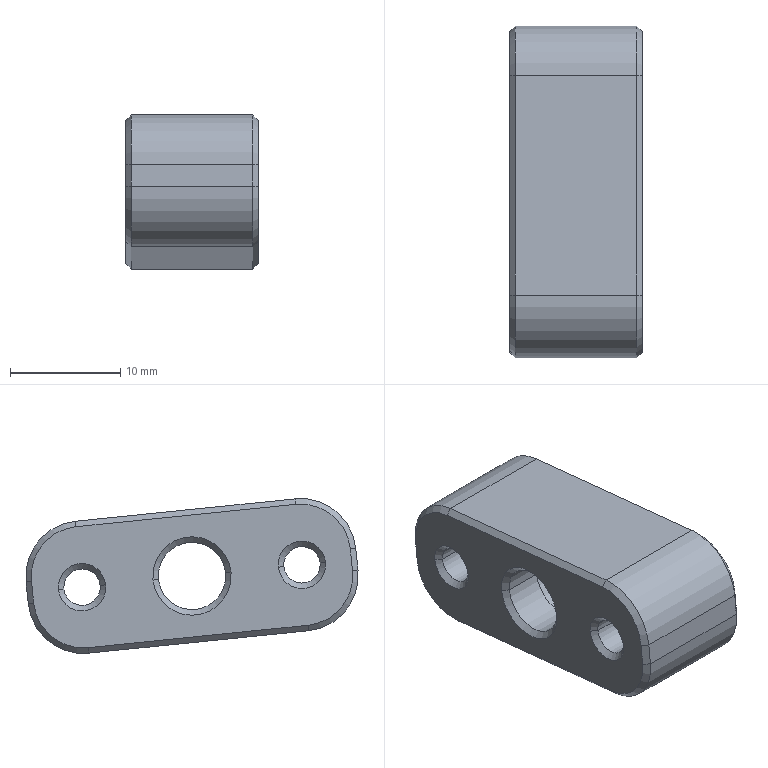Component | SolidWorks | 2018SOLIDWORKS1000000023-3 | 1 solid | 41 faces | box 12 x 30.1 x 14.01 mm | volume 3207 mm3 | plane 15 | cone 14 | cylinder 12 | commonest cylinder face diameters 3.3 x4 10 x4 9 x2 6.1 x2 | material 45 Steel
build123d program:
from build123d import *

# Parameters (mm, degrees)
SKETCH1_W           = 30
SKETCH1_H           = 12
BOSS_EXTRUDE1_DEPTH = 12
M4_TAPPED_HOLE1_D   = 3.3
SKETCH6_R           = 3.05
CUT_EXTRUDE3_DEPTH  = 21.125
FILLET1_R           = 5
SKETCH7_R           = 4.5
CUT_EXTRUDE4_DEPTH  = 8
CHAMFER2_SIZE       = 0.5


with BuildPart() as part:
    # Sketch1 → Boss-Extrude1 (new body)
    with BuildSketch(Plane.XY):
        Rectangle(SKETCH1_W, SKETCH1_H)
    extrude(amount=BOSS_EXTRUDE1_DEPTH)

    # M4 Tapped Hole1 (through all)
    with Locations(Plane.XY.offset(12)):
        with Locations((-10, 0), (10, 0)):
            Hole(M4_TAPPED_HOLE1_D / 2)

    # Sketch6 → Cut-Extrude3 (cut, through all)
    with BuildSketch(Plane.XY.offset(12)):
        Circle(SKETCH6_R)
    extrude(amount=-CUT_EXTRUDE3_DEPTH, mode=Mode.SUBTRACT)

    # Fillet1
    fillet1_edges = [part.edges().sort_by_distance(p)[0] for p in [
        (15, -6, 6),
        (-15, -6, 6),
        (-15, 6, 6),
        (15, 6, 6),
    ]]
    fillet(fillet1_edges, radius=FILLET1_R)

    # Sketch7 → Cut-Extrude4 (cut)
    with BuildSketch(Plane.XY.offset(12)):
        Circle(SKETCH7_R)
    extrude(amount=-CUT_EXTRUDE4_DEPTH, mode=Mode.SUBTRACT)

    # Chamfer2
    chamfer2_edges = [part.edges().sort_by_distance(p)[0] for p in [
        (11.65, 0, 0),
        (-8.35, 0, 0),
        (-3.05, 0, 0),
        (0, 6, 0),
        (0, 6, 12),
        (15, 0, 0),
        (0, -6, 0),
        (-15, 0, 0),
        (-13.536, -4.536, 0),
        (-13.536, 4.536, 0),
        (13.536, -4.536, 0),
        (13.536, 4.536, 0),
        (15, 0, 12),
        (-15, 0, 12),
        (0, -6, 12),
        (-13.536, -4.536, 12),
        (-13.536, 4.536, 12),
        (13.536, -4.536, 12),
        (13.536, 4.536, 12),
    ]]
    chamfer(chamfer2_edges, length=CHAMFER2_SIZE)


solid = part.part

# Placed as in the assembly
solid = solid.moved(Location((12.716, -65.924, 209.452), (-95.811, 90, 0)))